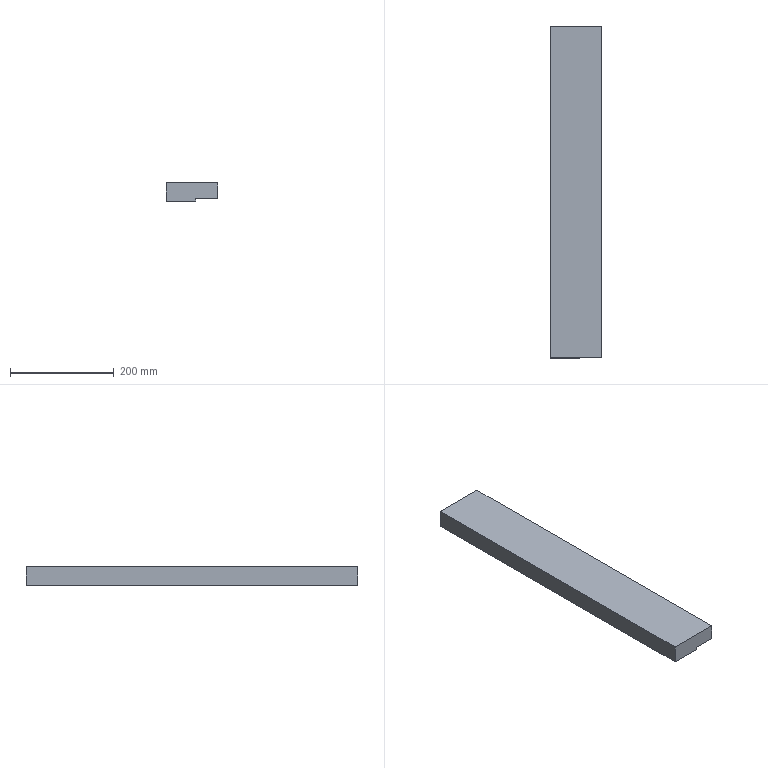Component | SolidWorks | JF21-80.1-1-3(_)-1-SOLID16-1 | 1 solid | 36 faces | box 100 x 640 x 35 mm | volume 2097027 mm3 | cylinder 14 | cone 14 | plane 8 | commonest cylinder face diameters 6.8 x12 10 x2
STEP:
#1=CARTESIAN_POINT('',(-12.648,-24.606,8.937));
#2=VERTEX_POINT('',#1);
#3=CARTESIAN_POINT('',(-12.648,-25.,8.937));
#4=VERTEX_POINT('',#3);
#5=CARTESIAN_POINT('',(-12.648,-24.803,8.937));
#6=DIRECTION('',(0.,-0.,1.));
#7=DIRECTION('',(0.,1.,0.));
#8=AXIS2_PLACEMENT_3D('',#5,#6,#7);
#9=CIRCLE('',#8,0.1969);
#10=EDGE_CURVE('',#2,#4,#9,.T.);
#11=ORIENTED_EDGE('',*,*,#10,.T.);
#12=CARTESIAN_POINT('',(-12.648,-25.,8.15));
#13=VERTEX_POINT('',#12);
#14=CARTESIAN_POINT('',(-12.648,-25.,8.15));
#15=DIRECTION('',(0.,0.,-1.));
#16=VECTOR('',#15,39.37);
#17=LINE('',#14,#16);
#18=EDGE_CURVE('',#4,#13,#17,.T.);
#19=ORIENTED_EDGE('',*,*,#18,.T.);
#20=CARTESIAN_POINT('',(-12.648,-24.606,8.15));
#21=VERTEX_POINT('',#20);
#22=CARTESIAN_POINT('',(-12.648,-24.803,8.15));
#23=DIRECTION('',(0.,-0.,1.));
#24=DIRECTION('',(0.,1.,0.));
#25=AXIS2_PLACEMENT_3D('',#22,#23,#24);
#26=CIRCLE('',#25,0.1969);
#27=EDGE_CURVE('',#21,#13,#26,.T.);
#28=ORIENTED_EDGE('',*,*,#27,.F.);
#29=CARTESIAN_POINT('',(-12.648,-24.606,8.15));
#30=DIRECTION('',(0.,0.,-1.));
#31=VECTOR('',#30,39.37);
#32=LINE('',#29,#31);
#33=EDGE_CURVE('',#2,#21,#32,.T.);
#34=ORIENTED_EDGE('',*,*,#33,.F.);
#35=EDGE_LOOP('',(#11,#19,#28,#34));
#36=FACE_OUTER_BOUND('',#35,.T.);
#37=CARTESIAN_POINT('',(-12.648,-24.803,8.15));
#38=DIRECTION('',(0.,0.,-1.));
#39=DIRECTION('',(0.,-1.,0.));
#40=AXIS2_PLACEMENT_3D('',#37,#38,#39);
#41=CYLINDRICAL_SURFACE('',#40,0.1969);
#42=ADVANCED_FACE('',(#36),#41,.F.);
#43=CARTESIAN_POINT('',(-12.648,-24.803,9.055));
#44=VERTEX_POINT('',#43);
#45=CARTESIAN_POINT('',(-12.648,-24.606,8.937));
#46=DIRECTION('',(0.,0.8572,-0.515));
#47=VECTOR('',#46,39.37);
#48=LINE('',#45,#47);
#49=EDGE_CURVE('',#44,#2,#48,.T.);
#50=ORIENTED_EDGE('',*,*,#49,.F.);
#51=CARTESIAN_POINT('',(-12.648,-25.,8.937));
#52=DIRECTION('',(0.,-0.8572,-0.515));
#53=VECTOR('',#52,39.37);
#54=LINE('',#51,#53);
#55=EDGE_CURVE('',#44,#4,#54,.T.);
#56=ORIENTED_EDGE('',*,*,#55,.T.);
#57=ORIENTED_EDGE('',*,*,#10,.F.);
#58=EDGE_LOOP('',(#50,#56,#57));
#59=FACE_OUTER_BOUND('',#58,.T.);
#60=CARTESIAN_POINT('',(-12.648,-24.803,8.937));
#61=DIRECTION('',(0.,0.,-1.));
#62=DIRECTION('',(0.,-1.,0.));
#63=AXIS2_PLACEMENT_3D('',#60,#61,#62);
#64=CONICAL_SURFACE('',#63,0.1969,1.03);
#65=ADVANCED_FACE('',(#59),#64,.F.);
#66=CARTESIAN_POINT('',(-12.648,-17.583,9.085));
#67=VERTEX_POINT('',#66);
#68=CARTESIAN_POINT('',(-12.648,-17.85,9.085));
#69=VERTEX_POINT('',#68);
#70=CARTESIAN_POINT('',(-12.648,-17.717,9.085));
#71=DIRECTION('',(0.,-0.,1.));
#72=DIRECTION('',(0.,1.,0.));
#73=AXIS2_PLACEMENT_3D('',#70,#71,#72);
#74=CIRCLE('',#73,0.1339);
#75=EDGE_CURVE('',#67,#69,#74,.T.);
#76=ORIENTED_EDGE('',*,*,#75,.T.);
#77=CARTESIAN_POINT('',(-12.648,-17.85,8.15));
#78=VERTEX_POINT('',#77);
#79=CARTESIAN_POINT('',(-12.648,-17.85,8.15));
#80=DIRECTION('',(0.,0.,-1.));
#81=VECTOR('',#80,39.37);
#82=LINE('',#79,#81);
#83=EDGE_CURVE('',#69,#78,#82,.T.);
#84=ORIENTED_EDGE('',*,*,#83,.T.);
#85=CARTESIAN_POINT('',(-12.648,-17.583,8.15));
#86=VERTEX_POINT('',#85);
#87=CARTESIAN_POINT('',(-12.648,-17.717,8.15));
#88=DIRECTION('',(0.,-0.,1.));
#89=DIRECTION('',(0.,1.,0.));
#90=AXIS2_PLACEMENT_3D('',#87,#88,#89);
#91=CIRCLE('',#90,0.1339);
#92=EDGE_CURVE('',#86,#78,#91,.T.);
#93=ORIENTED_EDGE('',*,*,#92,.F.);
#94=CARTESIAN_POINT('',(-12.648,-17.583,8.15));
#95=DIRECTION('',(0.,0.,-1.));
#96=VECTOR('',#95,39.37);
#97=LINE('',#94,#96);
#98=EDGE_CURVE('',#67,#86,#97,.T.);
#99=ORIENTED_EDGE('',*,*,#98,.F.);
#100=EDGE_LOOP('',(#76,#84,#93,#99));
#101=FACE_OUTER_BOUND('',#100,.T.);
#102=CARTESIAN_POINT('',(-12.648,-17.717,8.15));
#103=DIRECTION('',(0.,0.,-1.));
#104=DIRECTION('',(0.,-1.,0.));
#105=AXIS2_PLACEMENT_3D('',#102,#103,#104);
#106=CYLINDRICAL_SURFACE('',#105,0.1339);
#107=ADVANCED_FACE('',(#101),#106,.F.);
#108=CARTESIAN_POINT('',(-12.648,-17.717,9.165));
#109=VERTEX_POINT('',#108);
#110=CARTESIAN_POINT('',(-12.648,-17.583,9.085));
#111=DIRECTION('',(0.,0.8572,-0.515));
#112=VECTOR('',#111,39.37);
#113=LINE('',#110,#112);
#114=EDGE_CURVE('',#109,#67,#113,.T.);
#115=ORIENTED_EDGE('',*,*,#114,.F.);
#116=CARTESIAN_POINT('',(-12.648,-17.85,9.085));
#117=DIRECTION('',(0.,-0.8572,-0.515));
#118=VECTOR('',#117,39.37);
#119=LINE('',#116,#118);
#120=EDGE_CURVE('',#109,#69,#119,.T.);
#121=ORIENTED_EDGE('',*,*,#120,.T.);
#122=ORIENTED_EDGE('',*,*,#75,.F.);
#123=EDGE_LOOP('',(#115,#121,#122));
#124=FACE_OUTER_BOUND('',#123,.T.);
#125=CARTESIAN_POINT('',(-12.648,-17.717,9.085));
#126=DIRECTION('',(0.,0.,-1.));
#127=DIRECTION('',(0.,-1.,0.));
#128=AXIS2_PLACEMENT_3D('',#125,#126,#127);
#129=CONICAL_SURFACE('',#128,0.1339,1.03);
#130=ADVANCED_FACE('',(#124),#129,.F.);
#131=CARTESIAN_POINT('',(-12.648,-22.307,9.085));
#132=VERTEX_POINT('',#131);
#133=CARTESIAN_POINT('',(-12.648,-22.575,9.085));
#134=VERTEX_POINT('',#133);
#135=CARTESIAN_POINT('',(-12.648,-22.441,9.085));
#136=DIRECTION('',(0.,-0.,1.));
#137=DIRECTION('',(0.,1.,0.));
#138=AXIS2_PLACEMENT_3D('',#135,#136,#137);
#139=CIRCLE('',#138,0.1339);
#140=EDGE_CURVE('',#132,#134,#139,.T.);
#141=ORIENTED_EDGE('',*,*,#140,.T.);
#142=CARTESIAN_POINT('',(-12.648,-22.575,8.15));
#143=VERTEX_POINT('',#142);
#144=CARTESIAN_POINT('',(-12.648,-22.575,8.15));
#145=DIRECTION('',(0.,0.,-1.));
#146=VECTOR('',#145,39.37);
#147=LINE('',#144,#146);
#148=EDGE_CURVE('',#134,#143,#147,.T.);
#149=ORIENTED_EDGE('',*,*,#148,.T.);
#150=CARTESIAN_POINT('',(-12.648,-22.307,8.15));
#151=VERTEX_POINT('',#150);
#152=CARTESIAN_POINT('',(-12.648,-22.441,8.15));
#153=DIRECTION('',(0.,-0.,1.));
#154=DIRECTION('',(0.,1.,0.));
#155=AXIS2_PLACEMENT_3D('',#152,#153,#154);
#156=CIRCLE('',#155,0.1339);
#157=EDGE_CURVE('',#151,#143,#156,.T.);
#158=ORIENTED_EDGE('',*,*,#157,.F.);
#159=CARTESIAN_POINT('',(-12.648,-22.307,8.15));
#160=DIRECTION('',(0.,0.,-1.));
#161=VECTOR('',#160,39.37);
#162=LINE('',#159,#161);
#163=EDGE_CURVE('',#132,#151,#162,.T.);
#164=ORIENTED_EDGE('',*,*,#163,.F.);
#165=EDGE_LOOP('',(#141,#149,#158,#164));
#166=FACE_OUTER_BOUND('',#165,.T.);
#167=CARTESIAN_POINT('',(-12.648,-22.441,8.15));
#168=DIRECTION('',(0.,0.,-1.));
#169=DIRECTION('',(0.,-1.,0.));
#170=AXIS2_PLACEMENT_3D('',#167,#168,#169);
#171=CYLINDRICAL_SURFACE('',#170,0.1339);
#172=ADVANCED_FACE('',(#166),#171,.F.);
#173=CARTESIAN_POINT('',(-12.648,-22.441,9.165));
#174=VERTEX_POINT('',#173);
#175=CARTESIAN_POINT('',(-12.648,-22.307,9.085));
#176=DIRECTION('',(0.,0.8572,-0.515));
#177=VECTOR('',#176,39.37);
#178=LINE('',#175,#177);
#179=EDGE_CURVE('',#174,#132,#178,.T.);
#180=ORIENTED_EDGE('',*,*,#179,.F.);
#181=CARTESIAN_POINT('',(-12.648,-22.575,9.085));
#182=DIRECTION('',(0.,-0.8572,-0.515));
#183=VECTOR('',#182,39.37);
#184=LINE('',#181,#183);
#185=EDGE_CURVE('',#174,#134,#184,.T.);
#186=ORIENTED_EDGE('',*,*,#185,.T.);
#187=ORIENTED_EDGE('',*,*,#140,.F.);
#188=EDGE_LOOP('',(#180,#186,#187));
#189=FACE_OUTER_BOUND('',#188,.T.);
#190=CARTESIAN_POINT('',(-12.648,-22.441,9.085));
#191=DIRECTION('',(0.,0.,-1.));
#192=DIRECTION('',(0.,-1.,0.));
#193=AXIS2_PLACEMENT_3D('',#190,#191,#192);
#194=CONICAL_SURFACE('',#193,0.1339,1.03);
#195=ADVANCED_FACE('',(#189),#194,.F.);
#196=CARTESIAN_POINT('',(-12.648,-27.031,9.085));
#197=VERTEX_POINT('',#196);
#198=CARTESIAN_POINT('',(-12.648,-27.299,9.085));
#199=VERTEX_POINT('',#198);
#200=CARTESIAN_POINT('',(-12.648,-27.165,9.085));
#201=DIRECTION('',(0.,-0.,1.));
#202=DIRECTION('',(0.,1.,0.));
#203=AXIS2_PLACEMENT_3D('',#200,#201,#202);
#204=CIRCLE('',#203,0.1339);
#205=EDGE_CURVE('',#197,#199,#204,.T.);
#206=ORIENTED_EDGE('',*,*,#205,.T.);
#207=CARTESIAN_POINT('',(-12.648,-27.299,8.15));
#208=VERTEX_POINT('',#207);
#209=CARTESIAN_POINT('',(-12.648,-27.299,8.15));
#210=DIRECTION('',(0.,0.,-1.));
#211=VECTOR('',#210,39.37);
#212=LINE('',#209,#211);
#213=EDGE_CURVE('',#199,#208,#212,.T.);
#214=ORIENTED_EDGE('',*,*,#213,.T.);
#215=CARTESIAN_POINT('',(-12.648,-27.031,8.15));
#216=VERTEX_POINT('',#215);
#217=CARTESIAN_POINT('',(-12.648,-27.165,8.15));
#218=DIRECTION('',(0.,-0.,1.));
#219=DIRECTION('',(0.,1.,0.));
#220=AXIS2_PLACEMENT_3D('',#217,#218,#219);
#221=CIRCLE('',#220,0.1339);
#222=EDGE_CURVE('',#216,#208,#221,.T.);
#223=ORIENTED_EDGE('',*,*,#222,.F.);
#224=CARTESIAN_POINT('',(-12.648,-27.031,8.15));
#225=DIRECTION('',(0.,0.,-1.));
#226=VECTOR('',#225,39.37);
#227=LINE('',#224,#226);
#228=EDGE_CURVE('',#197,#216,#227,.T.);
#229=ORIENTED_EDGE('',*,*,#228,.F.);
#230=EDGE_LOOP('',(#206,#214,#223,#229));
#231=FACE_OUTER_BOUND('',#230,.T.);
#232=CARTESIAN_POINT('',(-12.648,-27.165,8.15));
#233=DIRECTION('',(0.,0.,-1.));
#234=DIRECTION('',(0.,-1.,0.));
#235=AXIS2_PLACEMENT_3D('',#232,#233,#234);
#236=CYLINDRICAL_SURFACE('',#235,0.1339);
#237=ADVANCED_FACE('',(#231),#236,.F.);
#238=CARTESIAN_POINT('',(-12.648,-27.165,9.165));
#239=VERTEX_POINT('',#238);
#240=CARTESIAN_POINT('',(-12.648,-27.031,9.085));
#241=DIRECTION('',(0.,0.8572,-0.515));
#242=VECTOR('',#241,39.37);
#243=LINE('',#240,#242);
#244=EDGE_CURVE('',#239,#197,#243,.T.);
#245=ORIENTED_EDGE('',*,*,#244,.F.);
#246=CARTESIAN_POINT('',(-12.648,-27.299,9.085));
#247=DIRECTION('',(0.,-0.8572,-0.515));
#248=VECTOR('',#247,39.37);
#249=LINE('',#246,#248);
#250=EDGE_CURVE('',#239,#199,#249,.T.);
#251=ORIENTED_EDGE('',*,*,#250,.T.);
#252=ORIENTED_EDGE('',*,*,#205,.F.);
#253=EDGE_LOOP('',(#245,#251,#252));
#254=FACE_OUTER_BOUND('',#253,.T.);
#255=CARTESIAN_POINT('',(-12.648,-27.165,9.085));
#256=DIRECTION('',(0.,0.,-1.));
#257=DIRECTION('',(0.,-1.,0.));
#258=AXIS2_PLACEMENT_3D('',#255,#256,#257);
#259=CONICAL_SURFACE('',#258,0.1339,1.03);
#260=ADVANCED_FACE('',(#254),#259,.F.);
#261=CARTESIAN_POINT('',(-12.648,-31.756,9.085));
#262=VERTEX_POINT('',#261);
#263=CARTESIAN_POINT('',(-12.648,-32.024,9.085));
#264=VERTEX_POINT('',#263);
#265=CARTESIAN_POINT('',(-12.648,-31.89,9.085));
#266=DIRECTION('',(0.,-0.,1.));
#267=DIRECTION('',(0.,1.,0.));
#268=AXIS2_PLACEMENT_3D('',#265,#266,#267);
#269=CIRCLE('',#268,0.1339);
#270=EDGE_CURVE('',#262,#264,#269,.T.);
#271=ORIENTED_EDGE('',*,*,#270,.T.);
#272=CARTESIAN_POINT('',(-12.648,-32.024,8.15));
#273=VERTEX_POINT('',#272);
#274=CARTESIAN_POINT('',(-12.648,-32.024,8.15));
#275=DIRECTION('',(0.,0.,-1.));
#276=VECTOR('',#275,39.37);
#277=LINE('',#274,#276);
#278=EDGE_CURVE('',#264,#273,#277,.T.);
#279=ORIENTED_EDGE('',*,*,#278,.T.);
#280=CARTESIAN_POINT('',(-12.648,-31.756,8.15));
#281=VERTEX_POINT('',#280);
#282=CARTESIAN_POINT('',(-12.648,-31.89,8.15));
#283=DIRECTION('',(0.,-0.,1.));
#284=DIRECTION('',(0.,1.,0.));
#285=AXIS2_PLACEMENT_3D('',#282,#283,#284);
#286=CIRCLE('',#285,0.1339);
#287=EDGE_CURVE('',#281,#273,#286,.T.);
#288=ORIENTED_EDGE('',*,*,#287,.F.);
#289=CARTESIAN_POINT('',(-12.648,-31.756,8.15));
#290=DIRECTION('',(0.,0.,-1.));
#291=VECTOR('',#290,39.37);
#292=LINE('',#289,#291);
#293=EDGE_CURVE('',#262,#281,#292,.T.);
#294=ORIENTED_EDGE('',*,*,#293,.F.);
#295=EDGE_LOOP('',(#271,#279,#288,#294));
#296=FACE_OUTER_BOUND('',#295,.T.);
#297=CARTESIAN_POINT('',(-12.648,-31.89,8.15));
#298=DIRECTION('',(0.,0.,-1.));
#299=DIRECTION('',(0.,-1.,0.));
#300=AXIS2_PLACEMENT_3D('',#297,#298,#299);
#301=CYLINDRICAL_SURFACE('',#300,0.1339);
#302=ADVANCED_FACE('',(#296),#301,.F.);
#303=CARTESIAN_POINT('',(-12.648,-31.89,9.165));
#304=VERTEX_POINT('',#303);
#305=CARTESIAN_POINT('',(-12.648,-31.756,9.085));
#306=DIRECTION('',(0.,0.8572,-0.515));
#307=VECTOR('',#306,39.37);
#308=LINE('',#305,#307);
#309=EDGE_CURVE('',#304,#262,#308,.T.);
#310=ORIENTED_EDGE('',*,*,#309,.F.);
#311=CARTESIAN_POINT('',(-12.648,-32.024,9.085));
#312=DIRECTION('',(0.,-0.8572,-0.515));
#313=VECTOR('',#312,39.37);
#314=LINE('',#311,#313);
#315=EDGE_CURVE('',#304,#264,#314,.T.);
#316=ORIENTED_EDGE('',*,*,#315,.T.);
#317=ORIENTED_EDGE('',*,*,#270,.F.);
#318=EDGE_LOOP('',(#310,#316,#317));
#319=FACE_OUTER_BOUND('',#318,.T.);
#320=CARTESIAN_POINT('',(-12.648,-31.89,9.085));
#321=DIRECTION('',(0.,0.,-1.));
#322=DIRECTION('',(0.,-1.,0.));
#323=AXIS2_PLACEMENT_3D('',#320,#321,#322);
#324=CONICAL_SURFACE('',#323,0.1339,1.03);
#325=ADVANCED_FACE('',(#319),#324,.F.);
#326=CARTESIAN_POINT('',(-12.648,-36.283,9.085));
#327=VERTEX_POINT('',#326);
#328=CARTESIAN_POINT('',(-12.648,-36.551,9.085));
#329=VERTEX_POINT('',#328);
#330=CARTESIAN_POINT('',(-12.648,-36.417,9.085));
#331=DIRECTION('',(0.,-0.,1.));
#332=DIRECTION('',(0.,1.,0.));
#333=AXIS2_PLACEMENT_3D('',#330,#331,#332);
#334=CIRCLE('',#333,0.1339);
#335=EDGE_CURVE('',#327,#329,#334,.T.);
#336=ORIENTED_EDGE('',*,*,#335,.T.);
#337=CARTESIAN_POINT('',(-12.648,-36.551,8.15));
#338=VERTEX_POINT('',#337);
#339=CARTESIAN_POINT('',(-12.648,-36.551,8.15));
#340=DIRECTION('',(0.,0.,-1.));
#341=VECTOR('',#340,39.37);
#342=LINE('',#339,#341);
#343=EDGE_CURVE('',#329,#338,#342,.T.);
#344=ORIENTED_EDGE('',*,*,#343,.T.);
#345=CARTESIAN_POINT('',(-12.648,-36.283,8.15));
#346=VERTEX_POINT('',#345);
#347=CARTESIAN_POINT('',(-12.648,-36.417,8.15));
#348=DIRECTION('',(0.,-0.,1.));
#349=DIRECTION('',(0.,1.,0.));
#350=AXIS2_PLACEMENT_3D('',#347,#348,#349);
#351=CIRCLE('',#350,0.1339);
#352=EDGE_CURVE('',#346,#338,#351,.T.);
#353=ORIENTED_EDGE('',*,*,#352,.F.);
#354=CARTESIAN_POINT('',(-12.648,-36.283,8.15));
#355=DIRECTION('',(0.,0.,-1.));
#356=VECTOR('',#355,39.37);
#357=LINE('',#354,#356);
#358=EDGE_CURVE('',#327,#346,#357,.T.);
#359=ORIENTED_EDGE('',*,*,#358,.F.);
#360=EDGE_LOOP('',(#336,#344,#353,#359));
#361=FACE_OUTER_BOUND('',#360,.T.);
#362=CARTESIAN_POINT('',(-12.648,-36.417,8.15));
#363=DIRECTION('',(0.,0.,-1.));
#364=DIRECTION('',(0.,-1.,0.));
#365=AXIS2_PLACEMENT_3D('',#362,#363,#364);
#366=CYLINDRICAL_SURFACE('',#365,0.1339);
#367=ADVANCED_FACE('',(#361),#366,.F.);
#368=CARTESIAN_POINT('',(-12.648,-36.417,9.165));
#369=VERTEX_POINT('',#368);
#370=CARTESIAN_POINT('',(-12.648,-36.283,9.085));
#371=DIRECTION('',(0.,0.8572,-0.515));
#372=VECTOR('',#371,39.37);
#373=LINE('',#370,#372);
#374=EDGE_CURVE('',#369,#327,#373,.T.);
#375=ORIENTED_EDGE('',*,*,#374,.F.);
#376=CARTESIAN_POINT('',(-12.648,-36.551,9.085));
#377=DIRECTION('',(0.,-0.8572,-0.515));
#378=VECTOR('',#377,39.37);
#379=LINE('',#376,#378);
#380=EDGE_CURVE('',#369,#329,#379,.T.);
#381=ORIENTED_EDGE('',*,*,#380,.T.);
#382=ORIENTED_EDGE('',*,*,#335,.F.);
#383=EDGE_LOOP('',(#375,#381,#382));
#384=FACE_OUTER_BOUND('',#383,.T.);
#385=CARTESIAN_POINT('',(-12.648,-36.417,9.085));
#386=DIRECTION('',(0.,0.,-1.));
#387=DIRECTION('',(0.,-1.,0.));
#388=AXIS2_PLACEMENT_3D('',#385,#386,#387);
#389=CONICAL_SURFACE('',#388,0.1339,1.03);
#390=ADVANCED_FACE('',(#384),#389,.F.);
#391=CARTESIAN_POINT('',(-12.648,-13.055,9.085));
#392=VERTEX_POINT('',#391);
#393=CARTESIAN_POINT('',(-12.648,-13.323,9.085));
#394=VERTEX_POINT('',#393);
#395=CARTESIAN_POINT('',(-12.648,-13.189,9.085));
#396=DIRECTION('',(0.,-0.,1.));
#397=DIRECTION('',(0.,1.,0.));
#398=AXIS2_PLACEMENT_3D('',#395,#396,#397);
#399=CIRCLE('',#398,0.1339);
#400=EDGE_CURVE('',#392,#394,#399,.T.);
#401=ORIENTED_EDGE('',*,*,#400,.T.);
#402=CARTESIAN_POINT('',(-12.648,-13.323,8.15));
#403=VERTEX_POINT('',#402);
#404=CARTESIAN_POINT('',(-12.648,-13.323,8.15));
#405=DIRECTION('',(0.,0.,-1.));
#406=VECTOR('',#405,39.37);
#407=LINE('',#404,#406);
#408=EDGE_CURVE('',#394,#403,#407,.T.);
#409=ORIENTED_EDGE('',*,*,#408,.T.);
#410=CARTESIAN_POINT('',(-12.648,-13.055,8.15));
#411=VERTEX_POINT('',#410);
#412=CARTESIAN_POINT('',(-12.648,-13.189,8.15));
#413=DIRECTION('',(0.,-0.,1.));
#414=DIRECTION('',(0.,1.,0.));
#415=AXIS2_PLACEMENT_3D('',#412,#413,#414);
#416=CIRCLE('',#415,0.1339);
#417=EDGE_CURVE('',#411,#403,#416,.T.);
#418=ORIENTED_EDGE('',*,*,#417,.F.);
#419=CARTESIAN_POINT('',(-12.648,-13.055,8.15));
#420=DIRECTION('',(0.,0.,-1.));
#421=VECTOR('',#420,39.37);
#422=LINE('',#419,#421);
#423=EDGE_CURVE('',#392,#411,#422,.T.);
#424=ORIENTED_EDGE('',*,*,#423,.F.);
#425=EDGE_LOOP('',(#401,#409,#418,#424));
#426=FACE_OUTER_BOUND('',#425,.T.);
#427=CARTESIAN_POINT('',(-12.648,-13.189,8.15));
#428=DIRECTION('',(0.,0.,-1.));
#429=DIRECTION('',(0.,-1.,0.));
#430=AXIS2_PLACEMENT_3D('',#427,#428,#429);
#431=CYLINDRICAL_SURFACE('',#430,0.1339);
#432=ADVANCED_FACE('',(#426),#431,.F.);
#433=CARTESIAN_POINT('',(-12.648,-13.189,9.165));
#434=VERTEX_POINT('',#433);
#435=CARTESIAN_POINT('',(-12.648,-13.055,9.085));
#436=DIRECTION('',(0.,0.8572,-0.515));
#437=VECTOR('',#436,39.37);
#438=LINE('',#435,#437);
#439=EDGE_CURVE('',#434,#392,#438,.T.);
#440=ORIENTED_EDGE('',*,*,#439,.F.);
#441=CARTESIAN_POINT('',(-12.648,-13.323,9.085));
#442=DIRECTION('',(0.,-0.8572,-0.515));
#443=VECTOR('',#442,39.37);
#444=LINE('',#441,#443);
#445=EDGE_CURVE('',#434,#394,#444,.T.);
#446=ORIENTED_EDGE('',*,*,#445,.T.);
#447=ORIENTED_EDGE('',*,*,#400,.F.);
#448=EDGE_LOOP('',(#440,#446,#447));
#449=FACE_OUTER_BOUND('',#448,.T.);
#450=CARTESIAN_POINT('',(-12.648,-13.189,9.085));
#451=DIRECTION('',(0.,0.,-1.));
#452=DIRECTION('',(0.,-1.,0.));
#453=AXIS2_PLACEMENT_3D('',#450,#451,#452);
#454=CONICAL_SURFACE('',#453,0.1339,1.03);
#455=ADVANCED_FACE('',(#449),#454,.F.);
#456=CARTESIAN_POINT('',(-13.484,-37.402,7.953));
#457=VERTEX_POINT('',#456);
#458=CARTESIAN_POINT('',(-15.748,-37.402,7.953));
#459=VERTEX_POINT('',#458);
#460=CARTESIAN_POINT('',(-13.484,-37.402,7.953));
#461=DIRECTION('',(-1.,0.,0.));
#462=VECTOR('',#461,39.37);
#463=LINE('',#460,#462);
#464=EDGE_CURVE('',#457,#459,#463,.T.);
#465=ORIENTED_EDGE('',*,*,#464,.T.);
#466=CARTESIAN_POINT('',(-15.748,-12.205,7.953));
#467=VERTEX_POINT('',#466);
#468=CARTESIAN_POINT('',(-15.748,-12.205,7.953));
#469=DIRECTION('',(0.,-1.,-0.));
#470=VECTOR('',#469,39.37);
#471=LINE('',#468,#470);
#472=EDGE_CURVE('',#467,#459,#471,.T.);
#473=ORIENTED_EDGE('',*,*,#472,.F.);
#474=CARTESIAN_POINT('',(-13.484,-12.205,7.953));
#475=VERTEX_POINT('',#474);
#476=CARTESIAN_POINT('',(-13.484,-12.205,7.953));
#477=DIRECTION('',(-1.,0.,0.));
#478=VECTOR('',#477,39.37);
#479=LINE('',#476,#478);
#480=EDGE_CURVE('',#475,#467,#479,.T.);
#481=ORIENTED_EDGE('',*,*,#480,.F.);
#482=CARTESIAN_POINT('',(-13.484,-12.205,7.953));
#483=DIRECTION('',(0.,-1.,-0.));
#484=VECTOR('',#483,39.37);
#485=LINE('',#482,#484);
#486=EDGE_CURVE('',#475,#457,#485,.T.);
#487=ORIENTED_EDGE('',*,*,#486,.T.);
#488=EDGE_LOOP('',(#465,#473,#481,#487));
#489=FACE_OUTER_BOUND('',#488,.T.);
#490=CARTESIAN_POINT('',(-13.484,-12.205,7.953));
#491=DIRECTION('',(0.,0.,-1.));
#492=DIRECTION('',(0.,-1.,-0.));
#493=AXIS2_PLACEMENT_3D('',#490,#491,#492);
#494=PLANE('',#493);
#495=ADVANCED_FACE('',(#489),#494,.T.);
#496=CARTESIAN_POINT('',(-13.484,-37.402,8.15));
#497=VERTEX_POINT('',#496);
#498=CARTESIAN_POINT('',(-13.484,-37.402,8.15));
#499=DIRECTION('',(0.,0.,-1.));
#500=VECTOR('',#499,39.37);
#501=LINE('',#498,#500);
#502=EDGE_CURVE('',#497,#457,#501,.T.);
#503=ORIENTED_EDGE('',*,*,#502,.T.);
#504=ORIENTED_EDGE('',*,*,#486,.F.);
#505=CARTESIAN_POINT('',(-13.484,-12.205,8.15));
#506=VERTEX_POINT('',#505);
#507=CARTESIAN_POINT('',(-13.484,-12.205,8.15));
#508=DIRECTION('',(0.,0.,-1.));
#509=VECTOR('',#508,39.37);
#510=LINE('',#507,#509);
#511=EDGE_CURVE('',#506,#475,#510,.T.);
#512=ORIENTED_EDGE('',*,*,#511,.F.);
#513=CARTESIAN_POINT('',(-13.484,-12.205,8.15));
#514=DIRECTION('',(0.,-1.,-0.));
#515=VECTOR('',#514,39.37);
#516=LINE('',#513,#515);
#517=EDGE_CURVE('',#506,#497,#516,.T.);
#518=ORIENTED_EDGE('',*,*,#517,.T.);
#519=EDGE_LOOP('',(#503,#504,#512,#518));
#520=FACE_OUTER_BOUND('',#519,.T.);
#521=CARTESIAN_POINT('',(-13.484,-12.205,8.15));
#522=DIRECTION('',(1.,0.,0.));
#523=DIRECTION('',(0.,0.,-1.));
#524=AXIS2_PLACEMENT_3D('',#521,#522,#523);
#525=PLANE('',#524);
#526=ADVANCED_FACE('',(#520),#525,.T.);
#527=ORIENTED_EDGE('',*,*,#27,.T.);
#528=CARTESIAN_POINT('',(-12.648,-24.803,8.15));
#529=DIRECTION('',(0.,-0.,1.));
#530=DIRECTION('',(0.,1.,0.));
#531=AXIS2_PLACEMENT_3D('',#528,#529,#530);
#532=CIRCLE('',#531,0.1969);
#533=EDGE_CURVE('',#13,#21,#532,.T.);
#534=ORIENTED_EDGE('',*,*,#533,.T.);
#535=EDGE_LOOP('',(#527,#534));
#536=FACE_BOUND('',#535,.T.);
#537=ORIENTED_EDGE('',*,*,#92,.T.);
#538=CARTESIAN_POINT('',(-12.648,-17.717,8.15));
#539=DIRECTION('',(0.,-0.,1.));
#540=DIRECTION('',(0.,1.,0.));
#541=AXIS2_PLACEMENT_3D('',#538,#539,#540);
#542=CIRCLE('',#541,0.1339);
#543=EDGE_CURVE('',#78,#86,#542,.T.);
#544=ORIENTED_EDGE('',*,*,#543,.T.);
#545=EDGE_LOOP('',(#537,#544));
#546=FACE_BOUND('',#545,.T.);
#547=ORIENTED_EDGE('',*,*,#157,.T.);
#548=CARTESIAN_POINT('',(-12.648,-22.441,8.15));
#549=DIRECTION('',(0.,-0.,1.));
#550=DIRECTION('',(0.,1.,0.));
#551=AXIS2_PLACEMENT_3D('',#548,#549,#550);
#552=CIRCLE('',#551,0.1339);
#553=EDGE_CURVE('',#143,#151,#552,.T.);
#554=ORIENTED_EDGE('',*,*,#553,.T.);
#555=EDGE_LOOP('',(#547,#554));
#556=FACE_BOUND('',#555,.T.);
#557=ORIENTED_EDGE('',*,*,#222,.T.);
#558=CARTESIAN_POINT('',(-12.648,-27.165,8.15));
#559=DIRECTION('',(0.,-0.,1.));
#560=DIRECTION('',(0.,1.,0.));
#561=AXIS2_PLACEMENT_3D('',#558,#559,#560);
#562=CIRCLE('',#561,0.1339);
#563=EDGE_CURVE('',#208,#216,#562,.T.);
#564=ORIENTED_EDGE('',*,*,#563,.T.);
#565=EDGE_LOOP('',(#557,#564));
#566=FACE_BOUND('',#565,.T.);
#567=ORIENTED_EDGE('',*,*,#287,.T.);
#568=CARTESIAN_POINT('',(-12.648,-31.89,8.15));
#569=DIRECTION('',(0.,-0.,1.));
#570=DIRECTION('',(0.,1.,0.));
#571=AXIS2_PLACEMENT_3D('',#568,#569,#570);
#572=CIRCLE('',#571,0.1339);
#573=EDGE_CURVE('',#273,#281,#572,.T.);
#574=ORIENTED_EDGE('',*,*,#573,.T.);
#575=EDGE_LOOP('',(#567,#574));
#576=FACE_BOUND('',#575,.T.);
#577=ORIENTED_EDGE('',*,*,#352,.T.);
#578=CARTESIAN_POINT('',(-12.648,-36.417,8.15));
#579=DIRECTION('',(0.,-0.,1.));
#580=DIRECTION('',(0.,1.,0.));
#581=AXIS2_PLACEMENT_3D('',#578,#579,#580);
#582=CIRCLE('',#581,0.1339);
#583=EDGE_CURVE('',#338,#346,#582,.T.);
#584=ORIENTED_EDGE('',*,*,#583,.T.);
#585=EDGE_LOOP('',(#577,#584));
#586=FACE_BOUND('',#585,.T.);
#587=ORIENTED_EDGE('',*,*,#417,.T.);
#588=CARTESIAN_POINT('',(-12.648,-13.189,8.15));
#589=DIRECTION('',(0.,-0.,1.));
#590=DIRECTION('',(0.,1.,0.));
#591=AXIS2_PLACEMENT_3D('',#588,#589,#590);
#592=CIRCLE('',#591,0.1339);
#593=EDGE_CURVE('',#403,#411,#592,.T.);
#594=ORIENTED_EDGE('',*,*,#593,.T.);
#595=EDGE_LOOP('',(#587,#594));
#596=FACE_BOUND('',#595,.T.);
#597=CARTESIAN_POINT('',(-11.811,-37.402,8.15));
#598=VERTEX_POINT('',#597);
#599=CARTESIAN_POINT('',(-11.811,-37.402,8.15));
#600=DIRECTION('',(-1.,0.,0.));
#601=VECTOR('',#600,39.37);
#602=LINE('',#599,#601);
#603=EDGE_CURVE('',#598,#497,#602,.T.);
#604=ORIENTED_EDGE('',*,*,#603,.T.);
#605=ORIENTED_EDGE('',*,*,#517,.F.);
#606=CARTESIAN_POINT('',(-11.811,-12.205,8.15));
#607=VERTEX_POINT('',#606);
#608=CARTESIAN_POINT('',(-11.811,-12.205,8.15));
#609=DIRECTION('',(-1.,0.,0.));
#610=VECTOR('',#609,39.37);
#611=LINE('',#608,#610);
#612=EDGE_CURVE('',#607,#506,#611,.T.);
#613=ORIENTED_EDGE('',*,*,#612,.F.);
#614=CARTESIAN_POINT('',(-11.811,-12.205,8.15));
#615=DIRECTION('',(0.,-1.,-0.));
#616=VECTOR('',#615,39.37);
#617=LINE('',#614,#616);
#618=EDGE_CURVE('',#607,#598,#617,.T.);
#619=ORIENTED_EDGE('',*,*,#618,.T.);
#620=EDGE_LOOP('',(#604,#605,#613,#619));
#621=FACE_OUTER_BOUND('',#620,.T.);
#622=CARTESIAN_POINT('',(-11.811,-12.205,8.15));
#623=DIRECTION('',(0.,0.,-1.));
#624=DIRECTION('',(0.,-1.,-0.));
#625=AXIS2_PLACEMENT_3D('',#622,#623,#624);
#626=PLANE('',#625);
#627=ADVANCED_FACE('',(#536,#546,#556,#566,#576,#586,#596,#621),#626,.T.);
#628=CARTESIAN_POINT('',(-11.811,-37.402,9.331));
#629=VERTEX_POINT('',#628);
#630=CARTESIAN_POINT('',(-11.811,-37.402,9.331));
#631=DIRECTION('',(0.,0.,-1.));
#632=VECTOR('',#631,39.37);
#633=LINE('',#630,#632);
#634=EDGE_CURVE('',#629,#598,#633,.T.);
#635=ORIENTED_EDGE('',*,*,#634,.T.);
#636=ORIENTED_EDGE('',*,*,#618,.F.);
#637=CARTESIAN_POINT('',(-11.811,-12.205,9.331));
#638=VERTEX_POINT('',#637);
#639=CARTESIAN_POINT('',(-11.811,-12.205,9.331));
#640=DIRECTION('',(0.,0.,-1.));
#641=VECTOR('',#640,39.37);
#642=LINE('',#639,#641);
#643=EDGE_CURVE('',#638,#607,#642,.T.);
#644=ORIENTED_EDGE('',*,*,#643,.F.);
#645=CARTESIAN_POINT('',(-11.811,-12.205,9.331));
#646=DIRECTION('',(0.,-1.,-0.));
#647=VECTOR('',#646,39.37);
#648=LINE('',#645,#647);
#649=EDGE_CURVE('',#638,#629,#648,.T.);
#650=ORIENTED_EDGE('',*,*,#649,.T.);
#651=EDGE_LOOP('',(#635,#636,#644,#650));
#652=FACE_OUTER_BOUND('',#651,.T.);
#653=CARTESIAN_POINT('',(-11.811,-12.205,9.331));
#654=DIRECTION('',(1.,0.,0.));
#655=DIRECTION('',(0.,0.,-1.));
#656=AXIS2_PLACEMENT_3D('',#653,#654,#655);
#657=PLANE('',#656);
#658=ADVANCED_FACE('',(#652),#657,.T.);
#659=CARTESIAN_POINT('',(-15.748,-37.402,9.331));
#660=VERTEX_POINT('',#659);
#661=CARTESIAN_POINT('',(-15.748,-37.402,9.331));
#662=DIRECTION('',(1.,0.,0.));
#663=VECTOR('',#662,39.37);
#664=LINE('',#661,#663);
#665=EDGE_CURVE('',#660,#629,#664,.T.);
#666=ORIENTED_EDGE('',*,*,#665,.T.);
#667=ORIENTED_EDGE('',*,*,#649,.F.);
#668=CARTESIAN_POINT('',(-15.748,-12.205,9.331));
#669=VERTEX_POINT('',#668);
#670=CARTESIAN_POINT('',(-15.748,-12.205,9.331));
#671=DIRECTION('',(1.,0.,0.));
#672=VECTOR('',#671,39.37);
#673=LINE('',#670,#672);
#674=EDGE_CURVE('',#669,#638,#673,.T.);
#675=ORIENTED_EDGE('',*,*,#674,.F.);
#676=CARTESIAN_POINT('',(-15.748,-12.205,9.331));
#677=DIRECTION('',(0.,-1.,-0.));
#678=VECTOR('',#677,39.37);
#679=LINE('',#676,#678);
#680=EDGE_CURVE('',#669,#660,#679,.T.);
#681=ORIENTED_EDGE('',*,*,#680,.T.);
#682=EDGE_LOOP('',(#666,#667,#675,#681));
#683=FACE_OUTER_BOUND('',#682,.T.);
#684=CARTESIAN_POINT('',(-15.748,-12.205,9.331));
#685=DIRECTION('',(0.,-0.,1.));
#686=DIRECTION('',(0.,1.,0.));
#687=AXIS2_PLACEMENT_3D('',#684,#685,#686);
#688=PLANE('',#687);
#689=ADVANCED_FACE('',(#683),#688,.T.);
#690=CARTESIAN_POINT('',(-15.748,-37.402,7.953));
#691=DIRECTION('',(0.,0.,1.));
#692=VECTOR('',#691,39.37);
#693=LINE('',#690,#692);
#694=EDGE_CURVE('',#459,#660,#693,.T.);
#695=ORIENTED_EDGE('',*,*,#694,.T.);
#696=ORIENTED_EDGE('',*,*,#680,.F.);
#697=CARTESIAN_POINT('',(-15.748,-12.205,7.953));
#698=DIRECTION('',(0.,0.,1.));
#699=VECTOR('',#698,39.37);
#700=LINE('',#697,#699);
#701=EDGE_CURVE('',#467,#669,#700,.T.);
#702=ORIENTED_EDGE('',*,*,#701,.F.);
#703=ORIENTED_EDGE('',*,*,#472,.T.);
#704=EDGE_LOOP('',(#695,#696,#702,#703));
#705=FACE_OUTER_BOUND('',#704,.T.);
#706=CARTESIAN_POINT('',(-15.748,-12.205,7.953));
#707=DIRECTION('',(-1.,0.,0.));
#708=DIRECTION('',(0.,0.,1.));
#709=AXIS2_PLACEMENT_3D('',#706,#707,#708);
#710=PLANE('',#709);
#711=ADVANCED_FACE('',(#705),#710,.T.);
#712=ORIENTED_EDGE('',*,*,#480,.T.);
#713=ORIENTED_EDGE('',*,*,#701,.T.);
#714=ORIENTED_EDGE('',*,*,#674,.T.);
#715=ORIENTED_EDGE('',*,*,#643,.T.);
#716=ORIENTED_EDGE('',*,*,#612,.T.);
#717=ORIENTED_EDGE('',*,*,#511,.T.);
#718=EDGE_LOOP('',(#712,#713,#714,#715,#716,#717));
#719=FACE_OUTER_BOUND('',#718,.T.);
#720=CARTESIAN_POINT('',(-15.748,-12.205,7.953));
#721=DIRECTION('',(0.,-1.,0.));
#722=DIRECTION('',(0.,0.,1.));
#723=AXIS2_PLACEMENT_3D('',#720,#721,#722);
#724=PLANE('',#723);
#725=ADVANCED_FACE('',(#719),#724,.F.);
#726=ORIENTED_EDGE('',*,*,#464,.F.);
#727=ORIENTED_EDGE('',*,*,#502,.F.);
#728=ORIENTED_EDGE('',*,*,#603,.F.);
#729=ORIENTED_EDGE('',*,*,#634,.F.);
#730=ORIENTED_EDGE('',*,*,#665,.F.);
#731=ORIENTED_EDGE('',*,*,#694,.F.);
#732=EDGE_LOOP('',(#726,#727,#728,#729,#730,#731));
#733=FACE_OUTER_BOUND('',#732,.T.);
#734=CARTESIAN_POINT('',(-15.748,-37.402,7.953));
#735=DIRECTION('',(0.,-1.,0.));
#736=DIRECTION('',(0.,0.,1.));
#737=AXIS2_PLACEMENT_3D('',#734,#735,#736);
#738=PLANE('',#737);
#739=ADVANCED_FACE('',(#733),#738,.T.);
#740=ORIENTED_EDGE('',*,*,#445,.F.);
#741=ORIENTED_EDGE('',*,*,#439,.T.);
#742=CARTESIAN_POINT('',(-12.648,-13.189,9.085));
#743=DIRECTION('',(0.,-0.,1.));
#744=DIRECTION('',(0.,1.,0.));
#745=AXIS2_PLACEMENT_3D('',#742,#743,#744);
#746=CIRCLE('',#745,0.1339);
#747=EDGE_CURVE('',#394,#392,#746,.T.);
#748=ORIENTED_EDGE('',*,*,#747,.F.);
#749=EDGE_LOOP('',(#740,#741,#748));
#750=FACE_OUTER_BOUND('',#749,.T.);
#751=CARTESIAN_POINT('',(-12.648,-13.189,9.085));
#752=DIRECTION('',(0.,0.,-1.));
#753=DIRECTION('',(0.,-1.,0.));
#754=AXIS2_PLACEMENT_3D('',#751,#752,#753);
#755=CONICAL_SURFACE('',#754,0.1339,1.03);
#756=ADVANCED_FACE('',(#750),#755,.F.);
#757=ORIENTED_EDGE('',*,*,#408,.F.);
#758=ORIENTED_EDGE('',*,*,#747,.T.);
#759=ORIENTED_EDGE('',*,*,#423,.T.);
#760=ORIENTED_EDGE('',*,*,#593,.F.);
#761=EDGE_LOOP('',(#757,#758,#759,#760));
#762=FACE_OUTER_BOUND('',#761,.T.);
#763=CARTESIAN_POINT('',(-12.648,-13.189,8.15));
#764=DIRECTION('',(0.,0.,-1.));
#765=DIRECTION('',(0.,-1.,0.));
#766=AXIS2_PLACEMENT_3D('',#763,#764,#765);
#767=CYLINDRICAL_SURFACE('',#766,0.1339);
#768=ADVANCED_FACE('',(#762),#767,.F.);
#769=ORIENTED_EDGE('',*,*,#380,.F.);
#770=ORIENTED_EDGE('',*,*,#374,.T.);
#771=CARTESIAN_POINT('',(-12.648,-36.417,9.085));
#772=DIRECTION('',(0.,-0.,1.));
#773=DIRECTION('',(0.,1.,0.));
#774=AXIS2_PLACEMENT_3D('',#771,#772,#773);
#775=CIRCLE('',#774,0.1339);
#776=EDGE_CURVE('',#329,#327,#775,.T.);
#777=ORIENTED_EDGE('',*,*,#776,.F.);
#778=EDGE_LOOP('',(#769,#770,#777));
#779=FACE_OUTER_BOUND('',#778,.T.);
#780=CARTESIAN_POINT('',(-12.648,-36.417,9.085));
#781=DIRECTION('',(0.,0.,-1.));
#782=DIRECTION('',(0.,-1.,0.));
#783=AXIS2_PLACEMENT_3D('',#780,#781,#782);
#784=CONICAL_SURFACE('',#783,0.1339,1.03);
#785=ADVANCED_FACE('',(#779),#784,.F.);
#786=ORIENTED_EDGE('',*,*,#343,.F.);
#787=ORIENTED_EDGE('',*,*,#776,.T.);
#788=ORIENTED_EDGE('',*,*,#358,.T.);
#789=ORIENTED_EDGE('',*,*,#583,.F.);
#790=EDGE_LOOP('',(#786,#787,#788,#789));
#791=FACE_OUTER_BOUND('',#790,.T.);
#792=CARTESIAN_POINT('',(-12.648,-36.417,8.15));
#793=DIRECTION('',(0.,0.,-1.));
#794=DIRECTION('',(0.,-1.,0.));
#795=AXIS2_PLACEMENT_3D('',#792,#793,#794);
#796=CYLINDRICAL_SURFACE('',#795,0.1339);
#797=ADVANCED_FACE('',(#791),#796,.F.);
#798=ORIENTED_EDGE('',*,*,#315,.F.);
#799=ORIENTED_EDGE('',*,*,#309,.T.);
#800=CARTESIAN_POINT('',(-12.648,-31.89,9.085));
#801=DIRECTION('',(0.,-0.,1.));
#802=DIRECTION('',(0.,1.,0.));
#803=AXIS2_PLACEMENT_3D('',#800,#801,#802);
#804=CIRCLE('',#803,0.1339);
#805=EDGE_CURVE('',#264,#262,#804,.T.);
#806=ORIENTED_EDGE('',*,*,#805,.F.);
#807=EDGE_LOOP('',(#798,#799,#806));
#808=FACE_OUTER_BOUND('',#807,.T.);
#809=CARTESIAN_POINT('',(-12.648,-31.89,9.085));
#810=DIRECTION('',(0.,0.,-1.));
#811=DIRECTION('',(0.,-1.,0.));
#812=AXIS2_PLACEMENT_3D('',#809,#810,#811);
#813=CONICAL_SURFACE('',#812,0.1339,1.03);
#814=ADVANCED_FACE('',(#808),#813,.F.);
#815=ORIENTED_EDGE('',*,*,#278,.F.);
#816=ORIENTED_EDGE('',*,*,#805,.T.);
#817=ORIENTED_EDGE('',*,*,#293,.T.);
#818=ORIENTED_EDGE('',*,*,#573,.F.);
#819=EDGE_LOOP('',(#815,#816,#817,#818));
#820=FACE_OUTER_BOUND('',#819,.T.);
#821=CARTESIAN_POINT('',(-12.648,-31.89,8.15));
#822=DIRECTION('',(0.,0.,-1.));
#823=DIRECTION('',(0.,-1.,0.));
#824=AXIS2_PLACEMENT_3D('',#821,#822,#823);
#825=CYLINDRICAL_SURFACE('',#824,0.1339);
#826=ADVANCED_FACE('',(#820),#825,.F.);
#827=ORIENTED_EDGE('',*,*,#250,.F.);
#828=ORIENTED_EDGE('',*,*,#244,.T.);
#829=CARTESIAN_POINT('',(-12.648,-27.165,9.085));
#830=DIRECTION('',(0.,-0.,1.));
#831=DIRECTION('',(0.,1.,0.));
#832=AXIS2_PLACEMENT_3D('',#829,#830,#831);
#833=CIRCLE('',#832,0.1339);
#834=EDGE_CURVE('',#199,#197,#833,.T.);
#835=ORIENTED_EDGE('',*,*,#834,.F.);
#836=EDGE_LOOP('',(#827,#828,#835));
#837=FACE_OUTER_BOUND('',#836,.T.);
#838=CARTESIAN_POINT('',(-12.648,-27.165,9.085));
#839=DIRECTION('',(0.,0.,-1.));
#840=DIRECTION('',(0.,-1.,0.));
#841=AXIS2_PLACEMENT_3D('',#838,#839,#840);
#842=CONICAL_SURFACE('',#841,0.1339,1.03);
#843=ADVANCED_FACE('',(#837),#842,.F.);
#844=ORIENTED_EDGE('',*,*,#213,.F.);
#845=ORIENTED_EDGE('',*,*,#834,.T.);
#846=ORIENTED_EDGE('',*,*,#228,.T.);
#847=ORIENTED_EDGE('',*,*,#563,.F.);
#848=EDGE_LOOP('',(#844,#845,#846,#847));
#849=FACE_OUTER_BOUND('',#848,.T.);
#850=CARTESIAN_POINT('',(-12.648,-27.165,8.15));
#851=DIRECTION('',(0.,0.,-1.));
#852=DIRECTION('',(0.,-1.,0.));
#853=AXIS2_PLACEMENT_3D('',#850,#851,#852);
#854=CYLINDRICAL_SURFACE('',#853,0.1339);
#855=ADVANCED_FACE('',(#849),#854,.F.);
#856=ORIENTED_EDGE('',*,*,#185,.F.);
#857=ORIENTED_EDGE('',*,*,#179,.T.);
#858=CARTESIAN_POINT('',(-12.648,-22.441,9.085));
#859=DIRECTION('',(0.,-0.,1.));
#860=DIRECTION('',(0.,1.,0.));
#861=AXIS2_PLACEMENT_3D('',#858,#859,#860);
#862=CIRCLE('',#861,0.1339);
#863=EDGE_CURVE('',#134,#132,#862,.T.);
#864=ORIENTED_EDGE('',*,*,#863,.F.);
#865=EDGE_LOOP('',(#856,#857,#864));
#866=FACE_OUTER_BOUND('',#865,.T.);
#867=CARTESIAN_POINT('',(-12.648,-22.441,9.085));
#868=DIRECTION('',(0.,0.,-1.));
#869=DIRECTION('',(0.,-1.,0.));
#870=AXIS2_PLACEMENT_3D('',#867,#868,#869);
#871=CONICAL_SURFACE('',#870,0.1339,1.03);
#872=ADVANCED_FACE('',(#866),#871,.F.);
#873=ORIENTED_EDGE('',*,*,#148,.F.);
#874=ORIENTED_EDGE('',*,*,#863,.T.);
#875=ORIENTED_EDGE('',*,*,#163,.T.);
#876=ORIENTED_EDGE('',*,*,#553,.F.);
#877=EDGE_LOOP('',(#873,#874,#875,#876));
#878=FACE_OUTER_BOUND('',#877,.T.);
#879=CARTESIAN_POINT('',(-12.648,-22.441,8.15));
#880=DIRECTION('',(0.,0.,-1.));
#881=DIRECTION('',(0.,-1.,0.));
#882=AXIS2_PLACEMENT_3D('',#879,#880,#881);
#883=CYLINDRICAL_SURFACE('',#882,0.1339);
#884=ADVANCED_FACE('',(#878),#883,.F.);
#885=ORIENTED_EDGE('',*,*,#120,.F.);
#886=ORIENTED_EDGE('',*,*,#114,.T.);
#887=CARTESIAN_POINT('',(-12.648,-17.717,9.085));
#888=DIRECTION('',(0.,-0.,1.));
#889=DIRECTION('',(0.,1.,0.));
#890=AXIS2_PLACEMENT_3D('',#887,#888,#889);
#891=CIRCLE('',#890,0.1339);
#892=EDGE_CURVE('',#69,#67,#891,.T.);
#893=ORIENTED_EDGE('',*,*,#892,.F.);
#894=EDGE_LOOP('',(#885,#886,#893));
#895=FACE_OUTER_BOUND('',#894,.T.);
#896=CARTESIAN_POINT('',(-12.648,-17.717,9.085));
#897=DIRECTION('',(0.,0.,-1.));
#898=DIRECTION('',(0.,-1.,0.));
#899=AXIS2_PLACEMENT_3D('',#896,#897,#898);
#900=CONICAL_SURFACE('',#899,0.1339,1.03);
#901=ADVANCED_FACE('',(#895),#900,.F.);
#902=ORIENTED_EDGE('',*,*,#83,.F.);
#903=ORIENTED_EDGE('',*,*,#892,.T.);
#904=ORIENTED_EDGE('',*,*,#98,.T.);
#905=ORIENTED_EDGE('',*,*,#543,.F.);
#906=EDGE_LOOP('',(#902,#903,#904,#905));
#907=FACE_OUTER_BOUND('',#906,.T.);
#908=CARTESIAN_POINT('',(-12.648,-17.717,8.15));
#909=DIRECTION('',(0.,0.,-1.));
#910=DIRECTION('',(0.,-1.,0.));
#911=AXIS2_PLACEMENT_3D('',#908,#909,#910);
#912=CYLINDRICAL_SURFACE('',#911,0.1339);
#913=ADVANCED_FACE('',(#907),#912,.F.);
#914=ORIENTED_EDGE('',*,*,#55,.F.);
#915=ORIENTED_EDGE('',*,*,#49,.T.);
#916=CARTESIAN_POINT('',(-12.648,-24.803,8.937));
#917=DIRECTION('',(0.,-0.,1.));
#918=DIRECTION('',(0.,1.,0.));
#919=AXIS2_PLACEMENT_3D('',#916,#917,#918);
#920=CIRCLE('',#919,0.1969);
#921=EDGE_CURVE('',#4,#2,#920,.T.);
#922=ORIENTED_EDGE('',*,*,#921,.F.);
#923=EDGE_LOOP('',(#914,#915,#922));
#924=FACE_OUTER_BOUND('',#923,.T.);
#925=CARTESIAN_POINT('',(-12.648,-24.803,8.937));
#926=DIRECTION('',(0.,0.,-1.));
#927=DIRECTION('',(0.,-1.,0.));
#928=AXIS2_PLACEMENT_3D('',#925,#926,#927);
#929=CONICAL_SURFACE('',#928,0.1969,1.03);
#930=ADVANCED_FACE('',(#924),#929,.F.);
#931=ORIENTED_EDGE('',*,*,#18,.F.);
#932=ORIENTED_EDGE('',*,*,#921,.T.);
#933=ORIENTED_EDGE('',*,*,#33,.T.);
#934=ORIENTED_EDGE('',*,*,#533,.F.);
#935=EDGE_LOOP('',(#931,#932,#933,#934));
#936=FACE_OUTER_BOUND('',#935,.T.);
#937=CARTESIAN_POINT('',(-12.648,-24.803,8.15));
#938=DIRECTION('',(0.,0.,-1.));
#939=DIRECTION('',(0.,-1.,0.));
#940=AXIS2_PLACEMENT_3D('',#937,#938,#939);
#941=CYLINDRICAL_SURFACE('',#940,0.1969);
#942=ADVANCED_FACE('',(#936),#941,.F.);
#943=CLOSED_SHELL('',(#42,#65,#107,#130,#172,#195,#237,#260,#302,#325,#367,#390,#432,#455,#495,#526,#627,#658,#689,#711,#725,#739,#756,#768,#785,#797,#814,#826,#843,#855,#872,#884,#901,#913,#930,#942));
#944=MANIFOLD_SOLID_BREP('',#943);
#945=CARTESIAN_POINT('',(0.,0.,0.));
#946=DIRECTION('',(0.,0.,1.));
#947=DIRECTION('',(1.,0.,0.));
#948=AXIS2_PLACEMENT_3D('',#945,#946,#947);
#949=(LENGTH_UNIT()NAMED_UNIT(*)SI_UNIT($,.METRE.));
#950=LENGTH_MEASURE_WITH_UNIT(LENGTH_MEASURE(0.0254),#949);
#951=DIMENSIONAL_EXPONENTS(1.,0.,0.,0.,0.,0.,0.);
#952=(CONVERSION_BASED_UNIT('',#950)LENGTH_UNIT()NAMED_UNIT(#951));
#953=UNCERTAINTY_MEASURE_WITH_UNIT(LENGTH_MEASURE(0.00001),#952,'','');
#954=(NAMED_UNIT(*)PLANE_ANGLE_UNIT()SI_UNIT($,.RADIAN.));
#955=(NAMED_UNIT(*)SI_UNIT($,.STERADIAN.)SOLID_ANGLE_UNIT());
#956=(GEOMETRIC_REPRESENTATION_CONTEXT(3)GLOBAL_UNCERTAINTY_ASSIGNED_CONTEXT((#953))GLOBAL_UNIT_ASSIGNED_CONTEXT((#952,#954,#955))REPRESENTATION_CONTEXT('',''));
#957=ADVANCED_BREP_SHAPE_REPRESENTATION('',(#944,#948),#956);
#958=COLOUR_RGB('',0.7922,0.8196,0.9333);
#959=FILL_AREA_STYLE_COLOUR('',#958);
#960=FILL_AREA_STYLE('',(#959));
#961=SURFACE_STYLE_FILL_AREA(#960);
#962=SURFACE_SIDE_STYLE('',(#961));
#963=SURFACE_STYLE_USAGE(.BOTH.,#962);
#964=PRESENTATION_STYLE_ASSIGNMENT((#963));
#965=STYLED_ITEM('',(#964),#944);
#966=(LENGTH_UNIT()NAMED_UNIT(*)SI_UNIT($,.METRE.));
#967=LENGTH_MEASURE_WITH_UNIT(LENGTH_MEASURE(0.0254),#966);
#968=DIMENSIONAL_EXPONENTS(1.,0.,0.,0.,0.,0.,0.);
#969=(CONVERSION_BASED_UNIT('',#967)LENGTH_UNIT()NAMED_UNIT(#968));
#970=UNCERTAINTY_MEASURE_WITH_UNIT(LENGTH_MEASURE(0.00001),#969,'','');
#971=(NAMED_UNIT(*)PLANE_ANGLE_UNIT()SI_UNIT($,.RADIAN.));
#972=(NAMED_UNIT(*)SI_UNIT($,.STERADIAN.)SOLID_ANGLE_UNIT());
#973=(GEOMETRIC_REPRESENTATION_CONTEXT(3)GLOBAL_UNCERTAINTY_ASSIGNED_CONTEXT((#970))GLOBAL_UNIT_ASSIGNED_CONTEXT((#969,#971,#972))REPRESENTATION_CONTEXT('',''));
#974=MECHANICAL_DESIGN_GEOMETRIC_PRESENTATION_REPRESENTATION('',(#965),#973);
#975=PRESENTATION_LAYER_ASSIGNMENT('','',(#965));